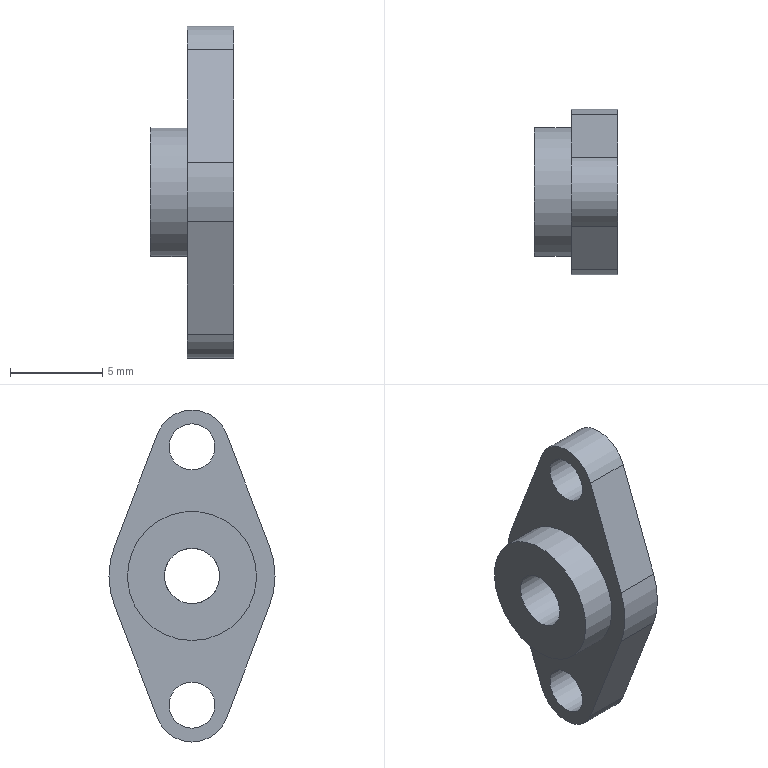Component | NX | EXT_CYLINDER_BODY_END_COVER | 1 solid | 15 faces | volume 294 mm3 | cylinder 8 | plane 7 | commonest cylinder face diameters 4 x2 9 x2 2.5 x2 7 x1 3 x1